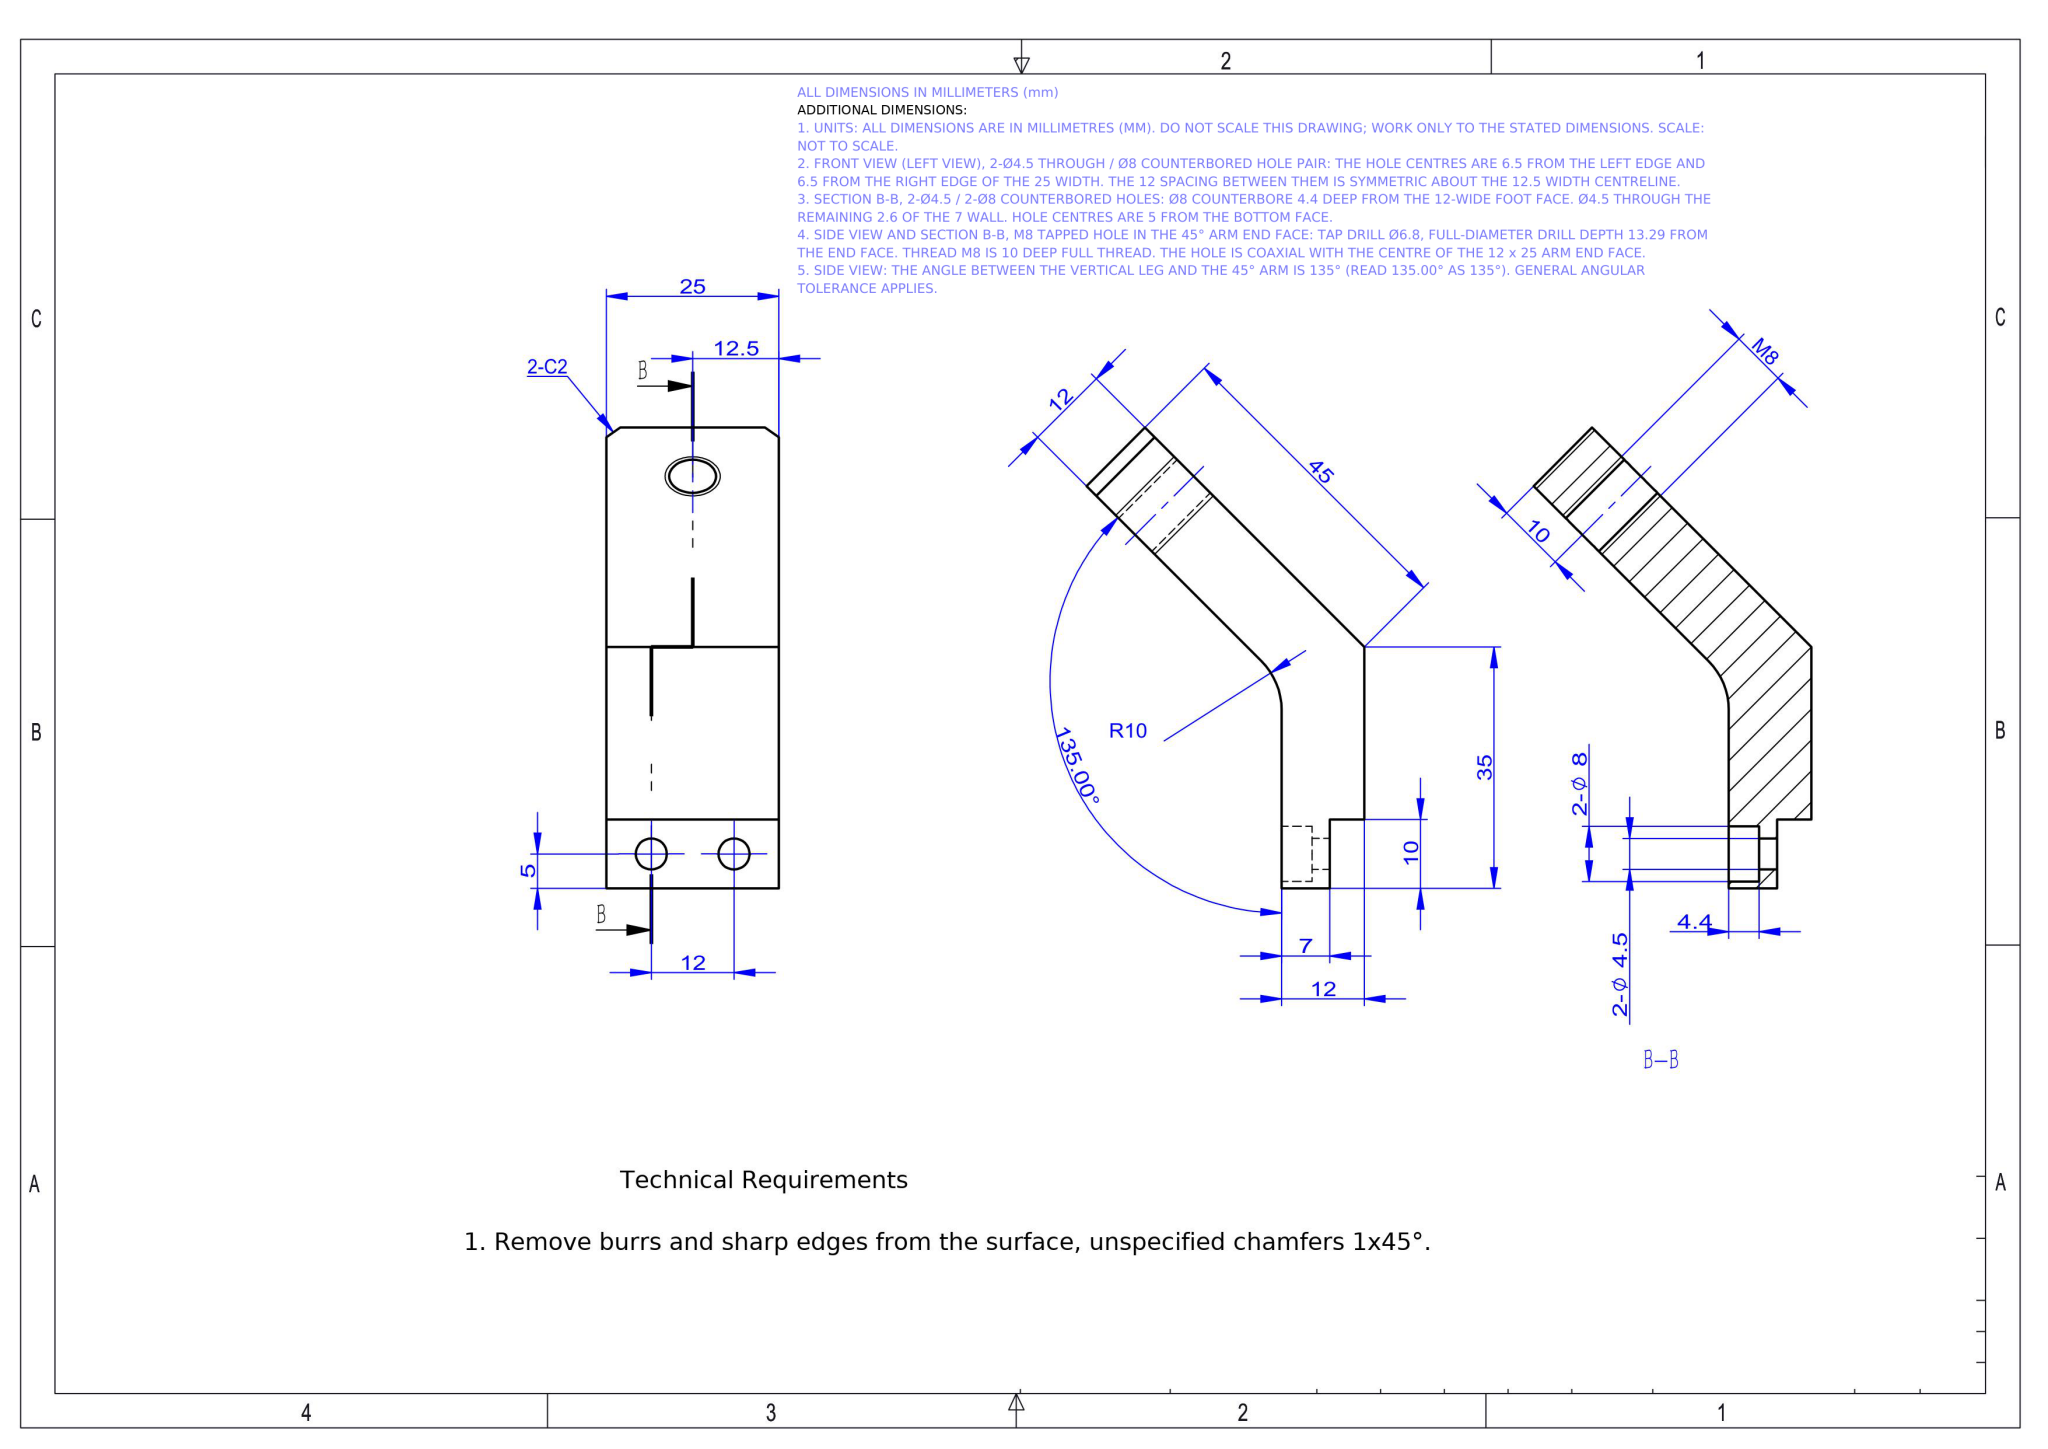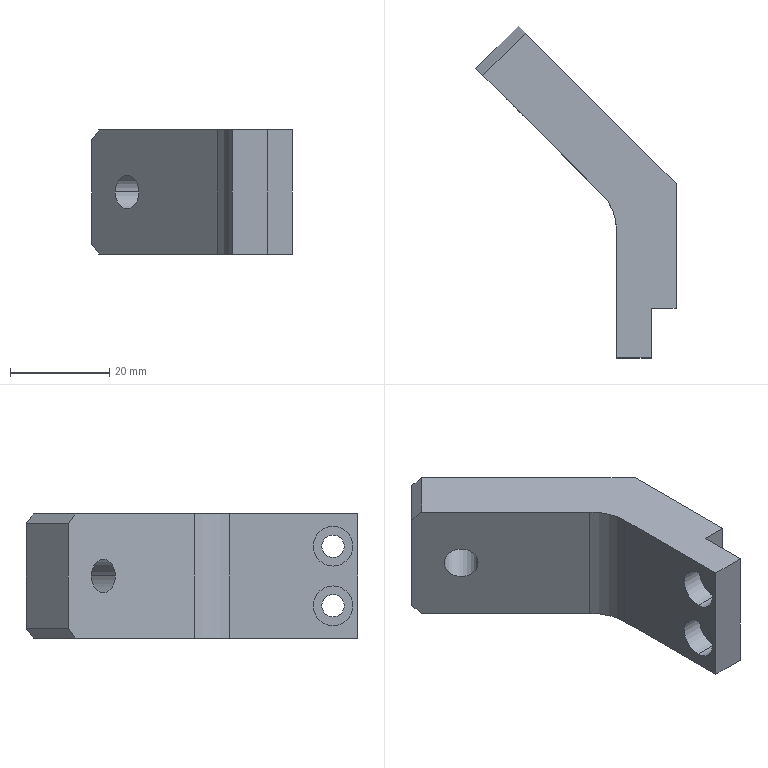Part | NX | mm | 295 | 1 solid | 25 faces | box 40.31 x 66.82 x 25 mm | volume 20304 mm3 | plane 14 | cylinder 11 | commonest cylinder face diameters 8 x4 4.5 x4 6.8 x2 20 x1
STEP:
#1=COLOUR_RGB('',0.7529,0.7529,0.7529);
#2=FILL_AREA_STYLE_COLOUR('',#1);
#3=FILL_AREA_STYLE('',(#2));
#4=SURFACE_STYLE_FILL_AREA(#3);
#5=SURFACE_SIDE_STYLE('',(#4));
#6=SURFACE_STYLE_USAGE(.BOTH.,#5);
#7=PRESENTATION_STYLE_ASSIGNMENT((#6));
#8=CARTESIAN_POINT('',(-30.83,13.859,12.5));
#9=VERTEX_POINT('',#8);
#10=CARTESIAN_POINT('',(-35.638,18.668,12.5));
#11=VERTEX_POINT('',#10);
#12=CARTESIAN_POINT('',(-33.234,16.263,12.5));
#13=DIRECTION('',(0.7071,0.7071,0.));
#14=DIRECTION('',(-0.7071,0.7071,0.));
#15=AXIS2_PLACEMENT_3D('',#12,#13,#14);
#16=CIRCLE('',#15,3.4);
#17=EDGE_CURVE('',#9,#11,#16,.T.);
#18=ORIENTED_EDGE('',*,*,#17,.F.);
#19=CARTESIAN_POINT('',(-22.345,22.345,12.5));
#20=VERTEX_POINT('',#19);
#21=CARTESIAN_POINT('',(-22.345,22.345,12.5));
#22=DIRECTION('',(0.7071,0.7071,0.));
#23=VECTOR('',#22,1000.);
#24=LINE('',#21,#23);
#25=EDGE_CURVE('',#9,#20,#24,.T.);
#26=ORIENTED_EDGE('',*,*,#25,.T.);
#27=CARTESIAN_POINT('',(-27.153,27.153,12.5));
#28=VERTEX_POINT('',#27);
#29=CARTESIAN_POINT('',(-24.749,24.749,12.5));
#30=DIRECTION('',(0.7071,0.7071,0.));
#31=DIRECTION('',(-0.7071,0.7071,0.));
#32=AXIS2_PLACEMENT_3D('',#29,#30,#31);
#33=CIRCLE('',#32,3.4);
#34=EDGE_CURVE('',#20,#28,#33,.T.);
#35=ORIENTED_EDGE('',*,*,#34,.T.);
#36=CARTESIAN_POINT('',(-27.153,27.153,12.5));
#37=DIRECTION('',(0.7071,0.7071,0.));
#38=VECTOR('',#37,1000.);
#39=LINE('',#36,#38);
#40=EDGE_CURVE('',#11,#28,#39,.T.);
#41=ORIENTED_EDGE('',*,*,#40,.F.);
#42=EDGE_LOOP('',(#18,#26,#35,#41));
#43=FACE_OUTER_BOUND('',#42,.T.);
#44=CARTESIAN_POINT('',(-24.749,24.749,12.5));
#45=DIRECTION('',(0.7071,0.7071,0.));
#46=DIRECTION('',(-0.7071,0.7071,0.));
#47=AXIS2_PLACEMENT_3D('',#44,#45,#46);
#48=CYLINDRICAL_SURFACE('',#47,3.4);
#49=ADVANCED_FACE('',(#43),#48,.F.);
#50=STYLED_ITEM('',(#7),#49);
#51=PRESENTATION_LAYER_ASSIGNMENT('','',(#50));
#52=COLOUR_RGB('',0.7529,0.7529,0.7529);
#53=FILL_AREA_STYLE_COLOUR('',#52);
#54=FILL_AREA_STYLE('',(#53));
#55=SURFACE_STYLE_FILL_AREA(#54);
#56=SURFACE_SIDE_STYLE('',(#55));
#57=SURFACE_STYLE_USAGE(.BOTH.,#56);
#58=PRESENTATION_STYLE_ASSIGNMENT((#57));
#59=CARTESIAN_POINT('',(-7.6,-30.,2.5));
#60=VERTEX_POINT('',#59);
#61=CARTESIAN_POINT('',(-7.6,-30.,10.5));
#62=VERTEX_POINT('',#61);
#63=CARTESIAN_POINT('',(-7.6,-30.,6.5));
#64=DIRECTION('',(-1.,0.,0.));
#65=DIRECTION('',(0.,0.,1.));
#66=AXIS2_PLACEMENT_3D('',#63,#64,#65);
#67=CIRCLE('',#66,4.);
#68=EDGE_CURVE('',#60,#62,#67,.T.);
#69=ORIENTED_EDGE('',*,*,#68,.F.);
#70=CARTESIAN_POINT('',(-12.,-30.,2.5));
#71=VERTEX_POINT('',#70);
#72=CARTESIAN_POINT('',(-12.,-30.,2.5));
#73=DIRECTION('',(-1.,0.,0.));
#74=VECTOR('',#73,1000.);
#75=LINE('',#72,#74);
#76=EDGE_CURVE('',#60,#71,#75,.T.);
#77=ORIENTED_EDGE('',*,*,#76,.T.);
#78=CARTESIAN_POINT('',(-12.,-30.,10.5));
#79=VERTEX_POINT('',#78);
#80=CARTESIAN_POINT('',(-12.,-30.,6.5));
#81=DIRECTION('',(-1.,0.,0.));
#82=DIRECTION('',(0.,0.,1.));
#83=AXIS2_PLACEMENT_3D('',#80,#81,#82);
#84=CIRCLE('',#83,4.);
#85=EDGE_CURVE('',#71,#79,#84,.T.);
#86=ORIENTED_EDGE('',*,*,#85,.T.);
#87=CARTESIAN_POINT('',(-12.,-30.,10.5));
#88=DIRECTION('',(-1.,0.,0.));
#89=VECTOR('',#88,1000.);
#90=LINE('',#87,#89);
#91=EDGE_CURVE('',#62,#79,#90,.T.);
#92=ORIENTED_EDGE('',*,*,#91,.F.);
#93=EDGE_LOOP('',(#69,#77,#86,#92));
#94=FACE_OUTER_BOUND('',#93,.T.);
#95=CARTESIAN_POINT('',(-12.,-30.,6.5));
#96=DIRECTION('',(-1.,0.,0.));
#97=DIRECTION('',(0.,0.,1.));
#98=AXIS2_PLACEMENT_3D('',#95,#96,#97);
#99=CYLINDRICAL_SURFACE('',#98,4.);
#100=ADVANCED_FACE('',(#94),#99,.F.);
#101=CARTESIAN_POINT('',(-5.,-30.,4.25));
#102=VERTEX_POINT('',#101);
#103=CARTESIAN_POINT('',(-5.,-30.,8.75));
#104=VERTEX_POINT('',#103);
#105=CARTESIAN_POINT('',(-5.,-30.,6.5));
#106=DIRECTION('',(-1.,0.,0.));
#107=DIRECTION('',(0.,0.,1.));
#108=AXIS2_PLACEMENT_3D('',#105,#106,#107);
#109=CIRCLE('',#108,2.25);
#110=EDGE_CURVE('',#102,#104,#109,.T.);
#111=ORIENTED_EDGE('',*,*,#110,.F.);
#112=CARTESIAN_POINT('',(-7.6,-30.,4.25));
#113=VERTEX_POINT('',#112);
#114=CARTESIAN_POINT('',(-12.,-30.,4.25));
#115=DIRECTION('',(-1.,0.,0.));
#116=VECTOR('',#115,1000.);
#117=LINE('',#114,#116);
#118=EDGE_CURVE('',#102,#113,#117,.T.);
#119=ORIENTED_EDGE('',*,*,#118,.T.);
#120=CARTESIAN_POINT('',(-7.6,-30.,8.75));
#121=VERTEX_POINT('',#120);
#122=CARTESIAN_POINT('',(-7.6,-30.,6.5));
#123=DIRECTION('',(-1.,0.,0.));
#124=DIRECTION('',(0.,0.,1.));
#125=AXIS2_PLACEMENT_3D('',#122,#123,#124);
#126=CIRCLE('',#125,2.25);
#127=EDGE_CURVE('',#113,#121,#126,.T.);
#128=ORIENTED_EDGE('',*,*,#127,.T.);
#129=CARTESIAN_POINT('',(-12.,-30.,8.75));
#130=DIRECTION('',(-1.,0.,0.));
#131=VECTOR('',#130,1000.);
#132=LINE('',#129,#131);
#133=EDGE_CURVE('',#104,#121,#132,.T.);
#134=ORIENTED_EDGE('',*,*,#133,.F.);
#135=EDGE_LOOP('',(#111,#119,#128,#134));
#136=FACE_OUTER_BOUND('',#135,.T.);
#137=CARTESIAN_POINT('',(-12.,-30.,6.5));
#138=DIRECTION('',(-1.,0.,0.));
#139=DIRECTION('',(0.,0.,1.));
#140=AXIS2_PLACEMENT_3D('',#137,#138,#139);
#141=CYLINDRICAL_SURFACE('',#140,2.25);
#142=ADVANCED_FACE('',(#136),#141,.F.);
#143=CARTESIAN_POINT('',(-7.6,-30.,14.5));
#144=VERTEX_POINT('',#143);
#145=CARTESIAN_POINT('',(-7.6,-30.,22.5));
#146=VERTEX_POINT('',#145);
#147=CARTESIAN_POINT('',(-7.6,-30.,18.5));
#148=DIRECTION('',(-1.,0.,0.));
#149=DIRECTION('',(0.,0.,1.));
#150=AXIS2_PLACEMENT_3D('',#147,#148,#149);
#151=CIRCLE('',#150,4.);
#152=EDGE_CURVE('',#144,#146,#151,.T.);
#153=ORIENTED_EDGE('',*,*,#152,.F.);
#154=CARTESIAN_POINT('',(-12.,-30.,14.5));
#155=VERTEX_POINT('',#154);
#156=CARTESIAN_POINT('',(-12.,-30.,14.5));
#157=DIRECTION('',(-1.,0.,0.));
#158=VECTOR('',#157,1000.);
#159=LINE('',#156,#158);
#160=EDGE_CURVE('',#144,#155,#159,.T.);
#161=ORIENTED_EDGE('',*,*,#160,.T.);
#162=CARTESIAN_POINT('',(-12.,-30.,22.5));
#163=VERTEX_POINT('',#162);
#164=CARTESIAN_POINT('',(-12.,-30.,18.5));
#165=DIRECTION('',(-1.,0.,0.));
#166=DIRECTION('',(0.,0.,1.));
#167=AXIS2_PLACEMENT_3D('',#164,#165,#166);
#168=CIRCLE('',#167,4.);
#169=EDGE_CURVE('',#155,#163,#168,.T.);
#170=ORIENTED_EDGE('',*,*,#169,.T.);
#171=CARTESIAN_POINT('',(-12.,-30.,22.5));
#172=DIRECTION('',(-1.,0.,0.));
#173=VECTOR('',#172,1000.);
#174=LINE('',#171,#173);
#175=EDGE_CURVE('',#146,#163,#174,.T.);
#176=ORIENTED_EDGE('',*,*,#175,.F.);
#177=EDGE_LOOP('',(#153,#161,#170,#176));
#178=FACE_OUTER_BOUND('',#177,.T.);
#179=CARTESIAN_POINT('',(-12.,-30.,18.5));
#180=DIRECTION('',(-1.,0.,0.));
#181=DIRECTION('',(0.,0.,1.));
#182=AXIS2_PLACEMENT_3D('',#179,#180,#181);
#183=CYLINDRICAL_SURFACE('',#182,4.);
#184=ADVANCED_FACE('',(#178),#183,.F.);
#185=CARTESIAN_POINT('',(-5.,-30.,16.25));
#186=VERTEX_POINT('',#185);
#187=CARTESIAN_POINT('',(-5.,-30.,20.75));
#188=VERTEX_POINT('',#187);
#189=CARTESIAN_POINT('',(-5.,-30.,18.5));
#190=DIRECTION('',(-1.,0.,0.));
#191=DIRECTION('',(0.,0.,1.));
#192=AXIS2_PLACEMENT_3D('',#189,#190,#191);
#193=CIRCLE('',#192,2.25);
#194=EDGE_CURVE('',#186,#188,#193,.T.);
#195=ORIENTED_EDGE('',*,*,#194,.F.);
#196=CARTESIAN_POINT('',(-7.6,-30.,16.25));
#197=VERTEX_POINT('',#196);
#198=CARTESIAN_POINT('',(-12.,-30.,16.25));
#199=DIRECTION('',(-1.,0.,0.));
#200=VECTOR('',#199,1000.);
#201=LINE('',#198,#200);
#202=EDGE_CURVE('',#186,#197,#201,.T.);
#203=ORIENTED_EDGE('',*,*,#202,.T.);
#204=CARTESIAN_POINT('',(-7.6,-30.,20.75));
#205=VERTEX_POINT('',#204);
#206=CARTESIAN_POINT('',(-7.6,-30.,18.5));
#207=DIRECTION('',(-1.,0.,0.));
#208=DIRECTION('',(0.,0.,1.));
#209=AXIS2_PLACEMENT_3D('',#206,#207,#208);
#210=CIRCLE('',#209,2.25);
#211=EDGE_CURVE('',#197,#205,#210,.T.);
#212=ORIENTED_EDGE('',*,*,#211,.T.);
#213=CARTESIAN_POINT('',(-12.,-30.,20.75));
#214=DIRECTION('',(-1.,0.,0.));
#215=VECTOR('',#214,1000.);
#216=LINE('',#213,#215);
#217=EDGE_CURVE('',#188,#205,#216,.T.);
#218=ORIENTED_EDGE('',*,*,#217,.F.);
#219=EDGE_LOOP('',(#195,#203,#212,#218));
#220=FACE_OUTER_BOUND('',#219,.T.);
#221=CARTESIAN_POINT('',(-12.,-30.,18.5));
#222=DIRECTION('',(-1.,0.,0.));
#223=DIRECTION('',(0.,0.,1.));
#224=AXIS2_PLACEMENT_3D('',#221,#222,#223);
#225=CYLINDRICAL_SURFACE('',#224,2.25);
#226=ADVANCED_FACE('',(#220),#225,.F.);
#227=CARTESIAN_POINT('',(-12.,-30.,6.5));
#228=DIRECTION('',(-1.,0.,0.));
#229=DIRECTION('',(0.,0.,1.));
#230=AXIS2_PLACEMENT_3D('',#227,#228,#229);
#231=CIRCLE('',#230,4.);
#232=EDGE_CURVE('',#79,#71,#231,.T.);
#233=ORIENTED_EDGE('',*,*,#232,.F.);
#234=ORIENTED_EDGE('',*,*,#85,.F.);
#235=EDGE_LOOP('',(#233,#234));
#236=FACE_BOUND('',#235,.T.);
#237=CARTESIAN_POINT('',(-12.,-30.,18.5));
#238=DIRECTION('',(-1.,0.,0.));
#239=DIRECTION('',(0.,0.,1.));
#240=AXIS2_PLACEMENT_3D('',#237,#238,#239);
#241=CIRCLE('',#240,4.);
#242=EDGE_CURVE('',#163,#155,#241,.T.);
#243=ORIENTED_EDGE('',*,*,#242,.F.);
#244=ORIENTED_EDGE('',*,*,#169,.F.);
#245=EDGE_LOOP('',(#243,#244));
#246=FACE_BOUND('',#245,.T.);
#247=CARTESIAN_POINT('',(-12.,-9.113,25.));
#248=VERTEX_POINT('',#247);
#249=CARTESIAN_POINT('',(-12.,-35.,25.));
#250=VERTEX_POINT('',#249);
#251=CARTESIAN_POINT('',(-12.,-0.,25.));
#252=DIRECTION('',(0.,-1.,0.));
#253=VECTOR('',#252,1000.);
#254=LINE('',#251,#253);
#255=EDGE_CURVE('',#248,#250,#254,.T.);
#256=ORIENTED_EDGE('',*,*,#255,.F.);
#257=CARTESIAN_POINT('',(-12.,-9.113,0.));
#258=VERTEX_POINT('',#257);
#259=CARTESIAN_POINT('',(-12.,-9.113,0.));
#260=DIRECTION('',(0.,0.,-1.));
#261=VECTOR('',#260,1000.);
#262=LINE('',#259,#261);
#263=EDGE_CURVE('',#248,#258,#262,.T.);
#264=ORIENTED_EDGE('',*,*,#263,.T.);
#265=CARTESIAN_POINT('',(-12.,-35.,0.));
#266=VERTEX_POINT('',#265);
#267=CARTESIAN_POINT('',(-12.,-0.,0.));
#268=DIRECTION('',(0.,-1.,0.));
#269=VECTOR('',#268,1000.);
#270=LINE('',#267,#269);
#271=EDGE_CURVE('',#258,#266,#270,.T.);
#272=ORIENTED_EDGE('',*,*,#271,.T.);
#273=CARTESIAN_POINT('',(-12.,-35.,25.));
#274=DIRECTION('',(0.,0.,-1.));
#275=VECTOR('',#274,1000.);
#276=LINE('',#273,#275);
#277=EDGE_CURVE('',#250,#266,#276,.T.);
#278=ORIENTED_EDGE('',*,*,#277,.F.);
#279=EDGE_LOOP('',(#256,#264,#272,#278));
#280=FACE_OUTER_BOUND('',#279,.T.);
#281=CARTESIAN_POINT('',(-12.,-0.,25.));
#282=DIRECTION('',(1.,0.,0.));
#283=DIRECTION('',(-0.,1.,0.));
#284=AXIS2_PLACEMENT_3D('',#281,#282,#283);
#285=PLANE('',#284);
#286=ADVANCED_FACE('',(#236,#246,#280),#285,.F.);
#287=CARTESIAN_POINT('',(-5.,-35.,0.));
#288=VERTEX_POINT('',#287);
#289=CARTESIAN_POINT('',(-5.,-35.,25.));
#290=VERTEX_POINT('',#289);
#291=CARTESIAN_POINT('',(-5.,-35.,0.));
#292=DIRECTION('',(0.,0.,1.));
#293=VECTOR('',#292,1000.);
#294=LINE('',#291,#293);
#295=EDGE_CURVE('',#288,#290,#294,.T.);
#296=ORIENTED_EDGE('',*,*,#295,.T.);
#297=CARTESIAN_POINT('',(0.,-35.,25.));
#298=DIRECTION('',(-1.,0.,0.));
#299=VECTOR('',#298,1000.);
#300=LINE('',#297,#299);
#301=EDGE_CURVE('',#290,#250,#300,.T.);
#302=ORIENTED_EDGE('',*,*,#301,.T.);
#303=ORIENTED_EDGE('',*,*,#277,.T.);
#304=CARTESIAN_POINT('',(0.,-35.,0.));
#305=DIRECTION('',(-1.,0.,0.));
#306=VECTOR('',#305,1000.);
#307=LINE('',#304,#306);
#308=EDGE_CURVE('',#288,#266,#307,.T.);
#309=ORIENTED_EDGE('',*,*,#308,.F.);
#310=EDGE_LOOP('',(#296,#302,#303,#309));
#311=FACE_OUTER_BOUND('',#310,.T.);
#312=CARTESIAN_POINT('',(0.,-35.,25.));
#313=DIRECTION('',(0.,-1.,0.));
#314=DIRECTION('',(0.,0.,-1.));
#315=AXIS2_PLACEMENT_3D('',#312,#313,#314);
#316=PLANE('',#315);
#317=ADVANCED_FACE('',(#311),#316,.T.);
#318=CARTESIAN_POINT('',(0.,-25.,0.));
#319=VERTEX_POINT('',#318);
#320=CARTESIAN_POINT('',(0.,-25.,25.));
#321=VERTEX_POINT('',#320);
#322=CARTESIAN_POINT('',(0.,-25.,0.));
#323=DIRECTION('',(0.,0.,1.));
#324=VECTOR('',#323,1000.);
#325=LINE('',#322,#324);
#326=EDGE_CURVE('',#319,#321,#325,.T.);
#327=ORIENTED_EDGE('',*,*,#326,.F.);
#328=CARTESIAN_POINT('',(0.,0.,0.));
#329=VERTEX_POINT('',#328);
#330=CARTESIAN_POINT('',(0.,0.,0.));
#331=DIRECTION('',(0.,-1.,0.));
#332=VECTOR('',#331,1000.);
#333=LINE('',#330,#332);
#334=EDGE_CURVE('',#329,#319,#333,.T.);
#335=ORIENTED_EDGE('',*,*,#334,.F.);
#336=CARTESIAN_POINT('',(0.,0.,25.));
#337=VERTEX_POINT('',#336);
#338=CARTESIAN_POINT('',(0.,0.,25.));
#339=DIRECTION('',(0.,0.,-1.));
#340=VECTOR('',#339,1000.);
#341=LINE('',#338,#340);
#342=EDGE_CURVE('',#337,#329,#341,.T.);
#343=ORIENTED_EDGE('',*,*,#342,.F.);
#344=CARTESIAN_POINT('',(0.,0.,25.));
#345=DIRECTION('',(0.,-1.,0.));
#346=VECTOR('',#345,1000.);
#347=LINE('',#344,#346);
#348=EDGE_CURVE('',#337,#321,#347,.T.);
#349=ORIENTED_EDGE('',*,*,#348,.T.);
#350=EDGE_LOOP('',(#327,#335,#343,#349));
#351=FACE_OUTER_BOUND('',#350,.T.);
#352=CARTESIAN_POINT('',(0.,0.,25.));
#353=DIRECTION('',(1.,0.,0.));
#354=DIRECTION('',(-0.,1.,0.));
#355=AXIS2_PLACEMENT_3D('',#352,#353,#354);
#356=PLANE('',#355);
#357=ADVANCED_FACE('',(#351),#356,.T.);
#358=CARTESIAN_POINT('',(-24.749,24.749,12.5));
#359=DIRECTION('',(0.7071,0.7071,0.));
#360=DIRECTION('',(-0.7071,0.7071,0.));
#361=AXIS2_PLACEMENT_3D('',#358,#359,#360);
#362=CIRCLE('',#361,3.4);
#363=EDGE_CURVE('',#28,#20,#362,.T.);
#364=ORIENTED_EDGE('',*,*,#363,.F.);
#365=ORIENTED_EDGE('',*,*,#34,.F.);
#366=EDGE_LOOP('',(#364,#365));
#367=FACE_BOUND('',#366,.T.);
#368=CARTESIAN_POINT('',(-30.406,30.406,-0.));
#369=VERTEX_POINT('',#368);
#370=CARTESIAN_POINT('',(-31.82,31.82,0.));
#371=DIRECTION('',(0.7071,-0.7071,0.));
#372=VECTOR('',#371,1000.);
#373=LINE('',#370,#372);
#374=EDGE_CURVE('',#369,#329,#373,.T.);
#375=ORIENTED_EDGE('',*,*,#374,.F.);
#376=CARTESIAN_POINT('',(-31.82,31.82,2.));
#377=VERTEX_POINT('',#376);
#378=CARTESIAN_POINT('',(-39.952,39.952,13.5));
#379=DIRECTION('',(-0.5,0.5,0.7071));
#380=VECTOR('',#379,1000.);
#381=LINE('',#378,#380);
#382=EDGE_CURVE('',#369,#377,#381,.T.);
#383=ORIENTED_EDGE('',*,*,#382,.T.);
#384=CARTESIAN_POINT('',(-31.82,31.82,23.));
#385=VERTEX_POINT('',#384);
#386=CARTESIAN_POINT('',(-31.82,31.82,25.));
#387=DIRECTION('',(0.,0.,-1.));
#388=VECTOR('',#387,1000.);
#389=LINE('',#386,#388);
#390=EDGE_CURVE('',#385,#377,#389,.T.);
#391=ORIENTED_EDGE('',*,*,#390,.F.);
#392=CARTESIAN_POINT('',(-30.406,30.406,25.));
#393=VERTEX_POINT('',#392);
#394=CARTESIAN_POINT('',(-31.113,31.113,24.));
#395=DIRECTION('',(0.5,-0.5,0.7071));
#396=VECTOR('',#395,1000.);
#397=LINE('',#394,#396);
#398=EDGE_CURVE('',#385,#393,#397,.T.);
#399=ORIENTED_EDGE('',*,*,#398,.T.);
#400=CARTESIAN_POINT('',(-31.82,31.82,25.));
#401=DIRECTION('',(0.7071,-0.7071,0.));
#402=VECTOR('',#401,1000.);
#403=LINE('',#400,#402);
#404=EDGE_CURVE('',#393,#337,#403,.T.);
#405=ORIENTED_EDGE('',*,*,#404,.T.);
#406=ORIENTED_EDGE('',*,*,#342,.T.);
#407=EDGE_LOOP('',(#375,#383,#391,#399,#405,#406));
#408=FACE_OUTER_BOUND('',#407,.T.);
#409=CARTESIAN_POINT('',(-31.82,31.82,25.));
#410=DIRECTION('',(0.7071,0.7071,0.));
#411=DIRECTION('',(-0.7071,0.7071,0.));
#412=AXIS2_PLACEMENT_3D('',#409,#410,#411);
#413=PLANE('',#412);
#414=ADVANCED_FACE('',(#367,#408),#413,.T.);
#415=ORIENTED_EDGE('',*,*,#390,.T.);
#416=CARTESIAN_POINT('',(-40.305,23.335,2.));
#417=VERTEX_POINT('',#416);
#418=CARTESIAN_POINT('',(-40.305,23.335,2.));
#419=DIRECTION('',(-0.7071,-0.7071,0.));
#420=VECTOR('',#419,1000.);
#421=LINE('',#418,#420);
#422=EDGE_CURVE('',#377,#417,#421,.T.);
#423=ORIENTED_EDGE('',*,*,#422,.T.);
#424=CARTESIAN_POINT('',(-40.305,23.335,23.));
#425=VERTEX_POINT('',#424);
#426=CARTESIAN_POINT('',(-40.305,23.335,25.));
#427=DIRECTION('',(0.,0.,-1.));
#428=VECTOR('',#427,1000.);
#429=LINE('',#426,#428);
#430=EDGE_CURVE('',#425,#417,#429,.T.);
#431=ORIENTED_EDGE('',*,*,#430,.F.);
#432=CARTESIAN_POINT('',(-31.82,31.82,23.));
#433=DIRECTION('',(0.7071,0.7071,0.));
#434=VECTOR('',#433,1000.);
#435=LINE('',#432,#434);
#436=EDGE_CURVE('',#425,#385,#435,.T.);
#437=ORIENTED_EDGE('',*,*,#436,.T.);
#438=EDGE_LOOP('',(#415,#423,#431,#437));
#439=FACE_OUTER_BOUND('',#438,.T.);
#440=CARTESIAN_POINT('',(-40.305,23.335,25.));
#441=DIRECTION('',(-0.7071,0.7071,0.));
#442=DIRECTION('',(-0.7071,-0.7071,0.));
#443=AXIS2_PLACEMENT_3D('',#440,#441,#442);
#444=PLANE('',#443);
#445=ADVANCED_FACE('',(#439),#444,.T.);
#446=CARTESIAN_POINT('',(-33.234,16.263,12.5));
#447=DIRECTION('',(0.7071,0.7071,0.));
#448=DIRECTION('',(-0.7071,0.7071,0.));
#449=AXIS2_PLACEMENT_3D('',#446,#447,#448);
#450=CIRCLE('',#449,3.4);
#451=EDGE_CURVE('',#11,#9,#450,.T.);
#452=ORIENTED_EDGE('',*,*,#451,.T.);
#453=ORIENTED_EDGE('',*,*,#17,.T.);
#454=EDGE_LOOP('',(#452,#453));
#455=FACE_BOUND('',#454,.T.);
#456=ORIENTED_EDGE('',*,*,#430,.T.);
#457=CARTESIAN_POINT('',(-38.891,21.92,0.));
#458=VERTEX_POINT('',#457);
#459=CARTESIAN_POINT('',(-38.891,21.92,0.));
#460=DIRECTION('',(0.5,-0.5,-0.7071));
#461=VECTOR('',#460,1000.);
#462=LINE('',#459,#461);
#463=EDGE_CURVE('',#417,#458,#462,.T.);
#464=ORIENTED_EDGE('',*,*,#463,.T.);
#465=CARTESIAN_POINT('',(-14.929,-2.042,0.));
#466=VERTEX_POINT('',#465);
#467=CARTESIAN_POINT('',(-40.305,23.335,0.));
#468=DIRECTION('',(0.7071,-0.7071,0.));
#469=VECTOR('',#468,1000.);
#470=LINE('',#467,#469);
#471=EDGE_CURVE('',#458,#466,#470,.T.);
#472=ORIENTED_EDGE('',*,*,#471,.T.);
#473=CARTESIAN_POINT('',(-14.929,-2.042,25.));
#474=VERTEX_POINT('',#473);
#475=CARTESIAN_POINT('',(-14.929,-2.042,25.));
#476=DIRECTION('',(0.,0.,1.));
#477=VECTOR('',#476,1000.);
#478=LINE('',#475,#477);
#479=EDGE_CURVE('',#466,#474,#478,.T.);
#480=ORIENTED_EDGE('',*,*,#479,.T.);
#481=CARTESIAN_POINT('',(-38.891,21.92,25.));
#482=VERTEX_POINT('',#481);
#483=CARTESIAN_POINT('',(-40.305,23.335,25.));
#484=DIRECTION('',(0.7071,-0.7071,0.));
#485=VECTOR('',#484,1000.);
#486=LINE('',#483,#485);
#487=EDGE_CURVE('',#482,#474,#486,.T.);
#488=ORIENTED_EDGE('',*,*,#487,.F.);
#489=CARTESIAN_POINT('',(-40.305,23.335,23.));
#490=DIRECTION('',(-0.5,0.5,-0.7071));
#491=VECTOR('',#490,1000.);
#492=LINE('',#489,#491);
#493=EDGE_CURVE('',#482,#425,#492,.T.);
#494=ORIENTED_EDGE('',*,*,#493,.T.);
#495=EDGE_LOOP('',(#456,#464,#472,#480,#488,#494));
#496=FACE_OUTER_BOUND('',#495,.T.);
#497=CARTESIAN_POINT('',(-40.305,23.335,25.));
#498=DIRECTION('',(0.7071,0.7071,0.));
#499=DIRECTION('',(-0.7071,0.7071,0.));
#500=AXIS2_PLACEMENT_3D('',#497,#498,#499);
#501=PLANE('',#500);
#502=ADVANCED_FACE('',(#455,#496),#501,.F.);
#503=ORIENTED_EDGE('',*,*,#301,.F.);
#504=CARTESIAN_POINT('',(-5.,-25.,25.));
#505=VERTEX_POINT('',#504);
#506=CARTESIAN_POINT('',(-5.,-35.,25.));
#507=DIRECTION('',(0.,-1.,0.));
#508=VECTOR('',#507,1000.);
#509=LINE('',#506,#508);
#510=EDGE_CURVE('',#505,#290,#509,.T.);
#511=ORIENTED_EDGE('',*,*,#510,.F.);
#512=CARTESIAN_POINT('',(0.,-25.,25.));
#513=DIRECTION('',(-1.,0.,0.));
#514=VECTOR('',#513,1000.);
#515=LINE('',#512,#514);
#516=EDGE_CURVE('',#321,#505,#515,.T.);
#517=ORIENTED_EDGE('',*,*,#516,.F.);
#518=ORIENTED_EDGE('',*,*,#348,.F.);
#519=ORIENTED_EDGE('',*,*,#404,.F.);
#520=CARTESIAN_POINT('',(-38.891,21.92,25.));
#521=DIRECTION('',(-0.7071,-0.7071,0.));
#522=VECTOR('',#521,1000.);
#523=LINE('',#520,#522);
#524=EDGE_CURVE('',#393,#482,#523,.T.);
#525=ORIENTED_EDGE('',*,*,#524,.T.);
#526=ORIENTED_EDGE('',*,*,#487,.T.);
#527=CARTESIAN_POINT('',(-22.,-9.113,25.));
#528=DIRECTION('',(0.,0.,-1.));
#529=DIRECTION('',(-1.,0.,0.));
#530=AXIS2_PLACEMENT_3D('',#527,#528,#529);
#531=CIRCLE('',#530,10.);
#532=EDGE_CURVE('',#474,#248,#531,.T.);
#533=ORIENTED_EDGE('',*,*,#532,.T.);
#534=ORIENTED_EDGE('',*,*,#255,.T.);
#535=EDGE_LOOP('',(#503,#511,#517,#518,#519,#525,#526,#533,#534));
#536=FACE_OUTER_BOUND('',#535,.T.);
#537=CARTESIAN_POINT('',(0.,0.,25.));
#538=DIRECTION('',(0.,0.,-1.));
#539=DIRECTION('',(-1.,0.,0.));
#540=AXIS2_PLACEMENT_3D('',#537,#538,#539);
#541=PLANE('',#540);
#542=ADVANCED_FACE('',(#536),#541,.F.);
#543=CARTESIAN_POINT('',(-5.,-25.,0.));
#544=VERTEX_POINT('',#543);
#545=CARTESIAN_POINT('',(-5.,-35.,0.));
#546=DIRECTION('',(0.,-1.,0.));
#547=VECTOR('',#546,1000.);
#548=LINE('',#545,#547);
#549=EDGE_CURVE('',#544,#288,#548,.T.);
#550=ORIENTED_EDGE('',*,*,#549,.T.);
#551=ORIENTED_EDGE('',*,*,#308,.T.);
#552=ORIENTED_EDGE('',*,*,#271,.F.);
#553=CARTESIAN_POINT('',(-22.,-9.113,0.));
#554=DIRECTION('',(0.,0.,1.));
#555=DIRECTION('',(-1.,0.,0.));
#556=AXIS2_PLACEMENT_3D('',#553,#554,#555);
#557=CIRCLE('',#556,10.);
#558=EDGE_CURVE('',#258,#466,#557,.T.);
#559=ORIENTED_EDGE('',*,*,#558,.T.);
#560=ORIENTED_EDGE('',*,*,#471,.F.);
#561=CARTESIAN_POINT('',(-30.406,30.406,0.));
#562=DIRECTION('',(0.7071,0.7071,0.));
#563=VECTOR('',#562,1000.);
#564=LINE('',#561,#563);
#565=EDGE_CURVE('',#458,#369,#564,.T.);
#566=ORIENTED_EDGE('',*,*,#565,.T.);
#567=ORIENTED_EDGE('',*,*,#374,.T.);
#568=ORIENTED_EDGE('',*,*,#334,.T.);
#569=CARTESIAN_POINT('',(0.,-25.,0.));
#570=DIRECTION('',(-1.,0.,0.));
#571=VECTOR('',#570,1000.);
#572=LINE('',#569,#571);
#573=EDGE_CURVE('',#319,#544,#572,.T.);
#574=ORIENTED_EDGE('',*,*,#573,.T.);
#575=EDGE_LOOP('',(#550,#551,#552,#559,#560,#566,#567,#568,#574));
#576=FACE_OUTER_BOUND('',#575,.T.);
#577=CARTESIAN_POINT('',(0.,0.,0.));
#578=DIRECTION('',(0.,0.,-1.));
#579=DIRECTION('',(-1.,0.,0.));
#580=AXIS2_PLACEMENT_3D('',#577,#578,#579);
#581=PLANE('',#580);
#582=ADVANCED_FACE('',(#576),#581,.T.);
#583=ORIENTED_EDGE('',*,*,#532,.F.);
#584=ORIENTED_EDGE('',*,*,#479,.F.);
#585=ORIENTED_EDGE('',*,*,#558,.F.);
#586=ORIENTED_EDGE('',*,*,#263,.F.);
#587=EDGE_LOOP('',(#583,#584,#585,#586));
#588=FACE_OUTER_BOUND('',#587,.T.);
#589=CARTESIAN_POINT('',(-22.,-9.113,25.));
#590=DIRECTION('',(0.,0.,1.));
#591=DIRECTION('',(1.,0.,0.));
#592=AXIS2_PLACEMENT_3D('',#589,#590,#591);
#593=CYLINDRICAL_SURFACE('',#592,10.);
#594=ADVANCED_FACE('',(#588),#593,.F.);
#595=ORIENTED_EDGE('',*,*,#463,.F.);
#596=ORIENTED_EDGE('',*,*,#422,.F.);
#597=ORIENTED_EDGE('',*,*,#382,.F.);
#598=ORIENTED_EDGE('',*,*,#565,.F.);
#599=EDGE_LOOP('',(#595,#596,#597,#598));
#600=FACE_OUTER_BOUND('',#599,.T.);
#601=CARTESIAN_POINT('',(-30.406,30.406,0.));
#602=DIRECTION('',(0.5,-0.5,0.7071));
#603=DIRECTION('',(0.7071,0.7071,0.));
#604=AXIS2_PLACEMENT_3D('',#601,#602,#603);
#605=PLANE('',#604);
#606=ADVANCED_FACE('',(#600),#605,.F.);
#607=ORIENTED_EDGE('',*,*,#493,.F.);
#608=ORIENTED_EDGE('',*,*,#524,.F.);
#609=ORIENTED_EDGE('',*,*,#398,.F.);
#610=ORIENTED_EDGE('',*,*,#436,.F.);
#611=EDGE_LOOP('',(#607,#608,#609,#610));
#612=FACE_OUTER_BOUND('',#611,.T.);
#613=CARTESIAN_POINT('',(-40.305,23.335,23.));
#614=DIRECTION('',(-0.5,0.5,0.7071));
#615=DIRECTION('',(-0.7071,-0.7071,0.));
#616=AXIS2_PLACEMENT_3D('',#613,#614,#615);
#617=PLANE('',#616);
#618=ADVANCED_FACE('',(#612),#617,.T.);
#619=CARTESIAN_POINT('',(-5.,-30.,6.5));
#620=DIRECTION('',(-1.,0.,0.));
#621=DIRECTION('',(0.,0.,1.));
#622=AXIS2_PLACEMENT_3D('',#619,#620,#621);
#623=CIRCLE('',#622,2.25);
#624=EDGE_CURVE('',#104,#102,#623,.T.);
#625=ORIENTED_EDGE('',*,*,#624,.T.);
#626=ORIENTED_EDGE('',*,*,#110,.T.);
#627=EDGE_LOOP('',(#625,#626));
#628=FACE_BOUND('',#627,.T.);
#629=CARTESIAN_POINT('',(-5.,-30.,18.5));
#630=DIRECTION('',(-1.,0.,0.));
#631=DIRECTION('',(0.,0.,1.));
#632=AXIS2_PLACEMENT_3D('',#629,#630,#631);
#633=CIRCLE('',#632,2.25);
#634=EDGE_CURVE('',#188,#186,#633,.T.);
#635=ORIENTED_EDGE('',*,*,#634,.T.);
#636=ORIENTED_EDGE('',*,*,#194,.T.);
#637=EDGE_LOOP('',(#635,#636));
#638=FACE_BOUND('',#637,.T.);
#639=ORIENTED_EDGE('',*,*,#510,.T.);
#640=ORIENTED_EDGE('',*,*,#295,.F.);
#641=ORIENTED_EDGE('',*,*,#549,.F.);
#642=CARTESIAN_POINT('',(-5.,-25.,0.));
#643=DIRECTION('',(0.,0.,1.));
#644=VECTOR('',#643,1000.);
#645=LINE('',#642,#644);
#646=EDGE_CURVE('',#544,#505,#645,.T.);
#647=ORIENTED_EDGE('',*,*,#646,.T.);
#648=EDGE_LOOP('',(#639,#640,#641,#647));
#649=FACE_OUTER_BOUND('',#648,.T.);
#650=CARTESIAN_POINT('',(-5.,-35.,0.));
#651=DIRECTION('',(-1.,0.,0.));
#652=DIRECTION('',(0.,0.,1.));
#653=AXIS2_PLACEMENT_3D('',#650,#651,#652);
#654=PLANE('',#653);
#655=ADVANCED_FACE('',(#628,#638,#649),#654,.F.);
#656=ORIENTED_EDGE('',*,*,#516,.T.);
#657=ORIENTED_EDGE('',*,*,#646,.F.);
#658=ORIENTED_EDGE('',*,*,#573,.F.);
#659=ORIENTED_EDGE('',*,*,#326,.T.);
#660=EDGE_LOOP('',(#656,#657,#658,#659));
#661=FACE_OUTER_BOUND('',#660,.T.);
#662=CARTESIAN_POINT('',(0.,-25.,0.));
#663=DIRECTION('',(0.,1.,0.));
#664=DIRECTION('',(0.,0.,1.));
#665=AXIS2_PLACEMENT_3D('',#662,#663,#664);
#666=PLANE('',#665);
#667=ADVANCED_FACE('',(#661),#666,.F.);
#668=ORIENTED_EDGE('',*,*,#25,.F.);
#669=ORIENTED_EDGE('',*,*,#451,.F.);
#670=ORIENTED_EDGE('',*,*,#40,.T.);
#671=ORIENTED_EDGE('',*,*,#363,.T.);
#672=EDGE_LOOP('',(#668,#669,#670,#671));
#673=FACE_OUTER_BOUND('',#672,.T.);
#674=CARTESIAN_POINT('',(-24.749,24.749,12.5));
#675=DIRECTION('',(0.7071,0.7071,0.));
#676=DIRECTION('',(-0.7071,0.7071,0.));
#677=AXIS2_PLACEMENT_3D('',#674,#675,#676);
#678=CYLINDRICAL_SURFACE('',#677,3.4);
#679=ADVANCED_FACE('',(#673),#678,.F.);
#680=ORIENTED_EDGE('',*,*,#202,.F.);
#681=ORIENTED_EDGE('',*,*,#634,.F.);
#682=ORIENTED_EDGE('',*,*,#217,.T.);
#683=CARTESIAN_POINT('',(-7.6,-30.,18.5));
#684=DIRECTION('',(-1.,0.,0.));
#685=DIRECTION('',(0.,0.,1.));
#686=AXIS2_PLACEMENT_3D('',#683,#684,#685);
#687=CIRCLE('',#686,2.25);
#688=EDGE_CURVE('',#205,#197,#687,.T.);
#689=ORIENTED_EDGE('',*,*,#688,.T.);
#690=EDGE_LOOP('',(#680,#681,#682,#689));
#691=FACE_OUTER_BOUND('',#690,.T.);
#692=CARTESIAN_POINT('',(-12.,-30.,18.5));
#693=DIRECTION('',(-1.,0.,0.));
#694=DIRECTION('',(0.,0.,1.));
#695=AXIS2_PLACEMENT_3D('',#692,#693,#694);
#696=CYLINDRICAL_SURFACE('',#695,2.25);
#697=ADVANCED_FACE('',(#691),#696,.F.);
#698=ORIENTED_EDGE('',*,*,#688,.F.);
#699=ORIENTED_EDGE('',*,*,#211,.F.);
#700=EDGE_LOOP('',(#698,#699));
#701=FACE_BOUND('',#700,.T.);
#702=CARTESIAN_POINT('',(-7.6,-30.,18.5));
#703=DIRECTION('',(-1.,0.,0.));
#704=DIRECTION('',(0.,0.,1.));
#705=AXIS2_PLACEMENT_3D('',#702,#703,#704);
#706=CIRCLE('',#705,4.);
#707=EDGE_CURVE('',#146,#144,#706,.T.);
#708=ORIENTED_EDGE('',*,*,#707,.T.);
#709=ORIENTED_EDGE('',*,*,#152,.T.);
#710=EDGE_LOOP('',(#708,#709));
#711=FACE_OUTER_BOUND('',#710,.T.);
#712=CARTESIAN_POINT('',(-7.6,-27.75,18.5));
#713=DIRECTION('',(1.,0.,0.));
#714=DIRECTION('',(0.,0.,-1.));
#715=AXIS2_PLACEMENT_3D('',#712,#713,#714);
#716=PLANE('',#715);
#717=ADVANCED_FACE('',(#701,#711),#716,.F.);
#718=ORIENTED_EDGE('',*,*,#160,.F.);
#719=ORIENTED_EDGE('',*,*,#707,.F.);
#720=ORIENTED_EDGE('',*,*,#175,.T.);
#721=ORIENTED_EDGE('',*,*,#242,.T.);
#722=EDGE_LOOP('',(#718,#719,#720,#721));
#723=FACE_OUTER_BOUND('',#722,.T.);
#724=CARTESIAN_POINT('',(-12.,-30.,18.5));
#725=DIRECTION('',(-1.,0.,0.));
#726=DIRECTION('',(0.,0.,1.));
#727=AXIS2_PLACEMENT_3D('',#724,#725,#726);
#728=CYLINDRICAL_SURFACE('',#727,4.);
#729=ADVANCED_FACE('',(#723),#728,.F.);
#730=ORIENTED_EDGE('',*,*,#118,.F.);
#731=ORIENTED_EDGE('',*,*,#624,.F.);
#732=ORIENTED_EDGE('',*,*,#133,.T.);
#733=CARTESIAN_POINT('',(-7.6,-30.,6.5));
#734=DIRECTION('',(-1.,0.,0.));
#735=DIRECTION('',(0.,0.,1.));
#736=AXIS2_PLACEMENT_3D('',#733,#734,#735);
#737=CIRCLE('',#736,2.25);
#738=EDGE_CURVE('',#121,#113,#737,.T.);
#739=ORIENTED_EDGE('',*,*,#738,.T.);
#740=EDGE_LOOP('',(#730,#731,#732,#739));
#741=FACE_OUTER_BOUND('',#740,.T.);
#742=CARTESIAN_POINT('',(-12.,-30.,6.5));
#743=DIRECTION('',(-1.,0.,0.));
#744=DIRECTION('',(0.,0.,1.));
#745=AXIS2_PLACEMENT_3D('',#742,#743,#744);
#746=CYLINDRICAL_SURFACE('',#745,2.25);
#747=ADVANCED_FACE('',(#741),#746,.F.);
#748=ORIENTED_EDGE('',*,*,#738,.F.);
#749=ORIENTED_EDGE('',*,*,#127,.F.);
#750=EDGE_LOOP('',(#748,#749));
#751=FACE_BOUND('',#750,.T.);
#752=CARTESIAN_POINT('',(-7.6,-30.,6.5));
#753=DIRECTION('',(-1.,0.,0.));
#754=DIRECTION('',(0.,0.,1.));
#755=AXIS2_PLACEMENT_3D('',#752,#753,#754);
#756=CIRCLE('',#755,4.);
#757=EDGE_CURVE('',#62,#60,#756,.T.);
#758=ORIENTED_EDGE('',*,*,#757,.T.);
#759=ORIENTED_EDGE('',*,*,#68,.T.);
#760=EDGE_LOOP('',(#758,#759));
#761=FACE_OUTER_BOUND('',#760,.T.);
#762=CARTESIAN_POINT('',(-7.6,-27.75,6.5));
#763=DIRECTION('',(1.,0.,0.));
#764=DIRECTION('',(0.,0.,-1.));
#765=AXIS2_PLACEMENT_3D('',#762,#763,#764);
#766=PLANE('',#765);
#767=ADVANCED_FACE('',(#751,#761),#766,.F.);
#768=ORIENTED_EDGE('',*,*,#76,.F.);
#769=ORIENTED_EDGE('',*,*,#757,.F.);
#770=ORIENTED_EDGE('',*,*,#91,.T.);
#771=ORIENTED_EDGE('',*,*,#232,.T.);
#772=EDGE_LOOP('',(#768,#769,#770,#771));
#773=FACE_OUTER_BOUND('',#772,.T.);
#774=CARTESIAN_POINT('',(-12.,-30.,6.5));
#775=DIRECTION('',(-1.,0.,0.));
#776=DIRECTION('',(0.,0.,1.));
#777=AXIS2_PLACEMENT_3D('',#774,#775,#776);
#778=CYLINDRICAL_SURFACE('',#777,4.);
#779=ADVANCED_FACE('',(#773),#778,.F.);
#780=CLOSED_SHELL('',(#100,#142,#184,#226,#49,#286,#317,#357,#414,#445,#502,#542,#582,#594,#606,#618,#655,#667,#679,#697,#717,#729,#747,#767,#779));
#781=MANIFOLD_SOLID_BREP('',#780);
#782=STYLED_ITEM('',(#58),#781);
#783=(LENGTH_UNIT()NAMED_UNIT(*)SI_UNIT(.MILLI.,.METRE.));
#784=UNCERTAINTY_MEASURE_WITH_UNIT(LENGTH_MEASURE(0.00001),#783,'','');
#785=(NAMED_UNIT(*)PLANE_ANGLE_UNIT()SI_UNIT($,.RADIAN.));
#786=(NAMED_UNIT(*)SI_UNIT($,.STERADIAN.)SOLID_ANGLE_UNIT());
#787=(GEOMETRIC_REPRESENTATION_CONTEXT(3)GLOBAL_UNCERTAINTY_ASSIGNED_CONTEXT((#784))GLOBAL_UNIT_ASSIGNED_CONTEXT((#783,#785,#786))REPRESENTATION_CONTEXT('',''));
#788=MECHANICAL_DESIGN_GEOMETRIC_PRESENTATION_REPRESENTATION('',(#782),#787);
#789=(LENGTH_UNIT()NAMED_UNIT(*)SI_UNIT(.MILLI.,.METRE.));
#790=UNCERTAINTY_MEASURE_WITH_UNIT(LENGTH_MEASURE(0.00001),#789,'','');
#791=(NAMED_UNIT(*)PLANE_ANGLE_UNIT()SI_UNIT($,.RADIAN.));
#792=(NAMED_UNIT(*)SI_UNIT($,.STERADIAN.)SOLID_ANGLE_UNIT());
#793=(GEOMETRIC_REPRESENTATION_CONTEXT(3)GLOBAL_UNCERTAINTY_ASSIGNED_CONTEXT((#790))GLOBAL_UNIT_ASSIGNED_CONTEXT((#789,#791,#792))REPRESENTATION_CONTEXT('',''));
#794=MECHANICAL_DESIGN_GEOMETRIC_PRESENTATION_REPRESENTATION('',(#50),#793);
#795=COLOUR_RGB('',0.7529,0.7529,0.7529);
#796=FILL_AREA_STYLE_COLOUR('',#795);
#797=FILL_AREA_STYLE('',(#796));
#798=SURFACE_STYLE_FILL_AREA(#797);
#799=SURFACE_SIDE_STYLE('',(#798));
#800=SURFACE_STYLE_USAGE(.BOTH.,#799);
#801=PRESENTATION_STYLE_ASSIGNMENT((#800));
#802=CARTESIAN_POINT('',(0.,0.,0.));
#803=DIRECTION('',(0.,0.,1.));
#804=DIRECTION('',(1.,0.,0.));
#805=AXIS2_PLACEMENT_3D('',#802,#803,#804);
#806=(LENGTH_UNIT()NAMED_UNIT(*)SI_UNIT(.MILLI.,.METRE.));
#807=UNCERTAINTY_MEASURE_WITH_UNIT(LENGTH_MEASURE(0.00001),#806,'','');
#808=(NAMED_UNIT(*)PLANE_ANGLE_UNIT()SI_UNIT($,.RADIAN.));
#809=(NAMED_UNIT(*)SI_UNIT($,.STERADIAN.)SOLID_ANGLE_UNIT());
#810=(GEOMETRIC_REPRESENTATION_CONTEXT(3)GLOBAL_UNCERTAINTY_ASSIGNED_CONTEXT((#807))GLOBAL_UNIT_ASSIGNED_CONTEXT((#806,#808,#809))REPRESENTATION_CONTEXT('',''));
#811=ADVANCED_BREP_SHAPE_REPRESENTATION('',(#781,#805),#810);
#812=STYLED_ITEM('',(#801),#811);
#813=PRESENTATION_LAYER_ASSIGNMENT('','',(#812));
#814=COLOUR_RGB('',0.7529,0.7529,0.7529);
#815=FILL_AREA_STYLE_COLOUR('',#814);
#816=FILL_AREA_STYLE('',(#815));
#817=SURFACE_STYLE_FILL_AREA(#816);
#818=SURFACE_SIDE_STYLE('',(#817));
#819=SURFACE_STYLE_USAGE(.BOTH.,#818);
#820=PRESENTATION_STYLE_ASSIGNMENT((#819));
#821=STYLED_ITEM('',(#820),#679);
#822=PRESENTATION_LAYER_ASSIGNMENT('','',(#821));
#823=(LENGTH_UNIT()NAMED_UNIT(*)SI_UNIT(.MILLI.,.METRE.));
#824=UNCERTAINTY_MEASURE_WITH_UNIT(LENGTH_MEASURE(0.00001),#823,'','');
#825=(NAMED_UNIT(*)PLANE_ANGLE_UNIT()SI_UNIT($,.RADIAN.));
#826=(NAMED_UNIT(*)SI_UNIT($,.STERADIAN.)SOLID_ANGLE_UNIT());
#827=(GEOMETRIC_REPRESENTATION_CONTEXT(3)GLOBAL_UNCERTAINTY_ASSIGNED_CONTEXT((#824))GLOBAL_UNIT_ASSIGNED_CONTEXT((#823,#825,#826))REPRESENTATION_CONTEXT('',''));
#828=MECHANICAL_DESIGN_GEOMETRIC_PRESENTATION_REPRESENTATION('',(#821),#827);
#829=PRESENTATION_LAYER_ASSIGNMENT('','',(#782));
#830=(LENGTH_UNIT()NAMED_UNIT(*)SI_UNIT(.MILLI.,.METRE.));
#831=UNCERTAINTY_MEASURE_WITH_UNIT(LENGTH_MEASURE(0.00001),#830,'','');
#832=(NAMED_UNIT(*)PLANE_ANGLE_UNIT()SI_UNIT($,.RADIAN.));
#833=(NAMED_UNIT(*)SI_UNIT($,.STERADIAN.)SOLID_ANGLE_UNIT());
#834=(GEOMETRIC_REPRESENTATION_CONTEXT(3)GLOBAL_UNCERTAINTY_ASSIGNED_CONTEXT((#831))GLOBAL_UNIT_ASSIGNED_CONTEXT((#830,#832,#833))REPRESENTATION_CONTEXT('',''));
#835=MECHANICAL_DESIGN_GEOMETRIC_PRESENTATION_REPRESENTATION('',(#812),#834);